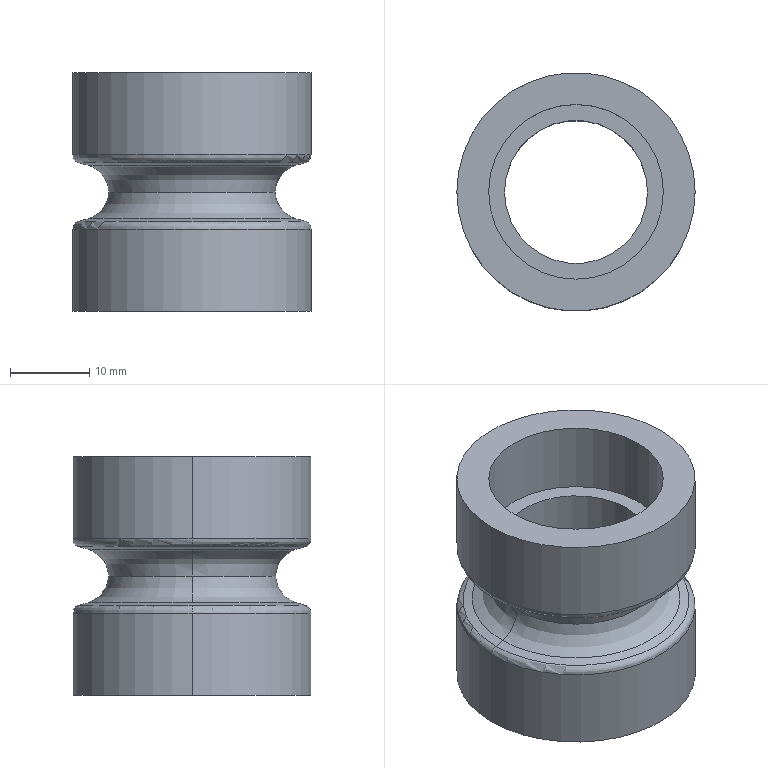Component | SolidWorks | JL001-03-03-1_JL001-03-03-002-1 | 1 solid | 26 faces | box 30 x 30 x 30 mm | volume 9084 mm3 | cylinder 10 | torus 8 | cone 4 | plane 4 | commonest cylinder face diameters 22 x4 30 x4 18 x2
build123d program:
from build123d import *

# Parameters (mm, degrees)
FILLET1_R = 1


with BuildPart() as part:
    # Sketch1 → Revolve1 (revolve)
    with BuildSketch(Plane.XY, mode=Mode.PRIVATE) as revolve1_sk:
        Polygon((11, 15), (15, 15), (15, -15), (11, -15), (11, -6), (9, -6), (9, 6), (11, 6), align=None)
    revolve(revolve1_sk.sketch.rotate(Axis((0, 0, 0), (0, -1, 0)), 90), axis=Axis((0, 0, 0), (0, -1, 0)))

    # Sketch2 → Cut-Revolve1 (revolve, cut)
    with BuildSketch(Plane.XY, mode=Mode.PRIVATE) as cut_revolve1_sk:
        with BuildLine():
            Line((13.094, 3.381), (16, 4.159))
            Line((16, 4.159), (16, -4.159))
            Line((16, -4.159), (13.094, -3.381))
            ThreePointArc((13.094, -3.381), (10.5, 0), (13.094, 3.381))
        make_face()
    revolve(cut_revolve1_sk.sketch.rotate(Axis((0, 0, 0), (0, -1, 0)), 90), axis=Axis((0, 0, 0), (0, -1, 0)), mode=Mode.SUBTRACT)

    # Fillet1
    fillet1_edges = [part.edges().sort_by_distance(p)[0] for p in [
        (0, -3.891, -15),
        (0, 3.891, -15),
    ]]
    fillet(fillet1_edges, radius=FILLET1_R)


solid = part.part

# Placed as in the assembly
solid = solid.moved(Location((15, 27.5, 40.5), (90, 0, 0)))
STEP:
#1=COLOUR_RGB('',0.7922,0.8196,0.9333);
#2=FILL_AREA_STYLE_COLOUR('',#1);
#3=FILL_AREA_STYLE('',(#2));
#4=SURFACE_STYLE_FILL_AREA(#3);
#5=SURFACE_SIDE_STYLE('',(#4));
#6=SURFACE_STYLE_USAGE(.BOTH.,#5);
#7=PRESENTATION_STYLE_ASSIGNMENT((#6));
#8=CARTESIAN_POINT('',(0.07503,1.083,1.728));
#9=VERTEX_POINT('',#8);
#10=CARTESIAN_POINT('',(0.1772,1.083,1.594));
#11=VERTEX_POINT('',#10);
#12=CARTESIAN_POINT('',(0.03937,1.083,1.594));
#13=DIRECTION('',(-0.,1.,0.));
#14=DIRECTION('',(-1.,0.,0.));
#15=AXIS2_PLACEMENT_3D('',#12,#13,#14);
#16=CIRCLE('',#15,0.1378);
#17=EDGE_CURVE('',#9,#11,#16,.T.);
#18=ORIENTED_EDGE('',*,*,#17,.T.);
#19=CARTESIAN_POINT('',(1.004,1.083,1.594));
#20=VERTEX_POINT('',#19);
#21=CARTESIAN_POINT('',(0.5906,1.083,1.594));
#22=DIRECTION('',(0.,0.,1.));
#23=DIRECTION('',(1.,0.,0.));
#24=AXIS2_PLACEMENT_3D('',#21,#22,#23);
#25=CIRCLE('',#24,0.4134);
#26=EDGE_CURVE('',#11,#20,#25,.T.);
#27=ORIENTED_EDGE('',*,*,#26,.T.);
#28=CARTESIAN_POINT('',(1.106,1.083,1.728));
#29=VERTEX_POINT('',#28);
#30=CARTESIAN_POINT('',(1.142,1.083,1.594));
#31=DIRECTION('',(0.,-1.,0.));
#32=DIRECTION('',(1.,0.,0.));
#33=AXIS2_PLACEMENT_3D('',#30,#31,#32);
#34=CIRCLE('',#33,0.1378);
#35=EDGE_CURVE('',#29,#20,#34,.T.);
#36=ORIENTED_EDGE('',*,*,#35,.F.);
#37=CARTESIAN_POINT('',(0.5906,1.083,1.728));
#38=DIRECTION('',(0.,0.,1.));
#39=DIRECTION('',(-1.,-0.,0.));
#40=AXIS2_PLACEMENT_3D('',#37,#38,#39);
#41=CIRCLE('',#40,0.5155);
#42=EDGE_CURVE('',#9,#29,#41,.T.);
#43=ORIENTED_EDGE('',*,*,#42,.F.);
#44=EDGE_LOOP('',(#18,#27,#36,#43));
#45=FACE_OUTER_BOUND('',#44,.T.);
#46=CARTESIAN_POINT('',(0.5906,1.083,1.594));
#47=DIRECTION('',(0.,0.,1.));
#48=DIRECTION('',(-1.,-0.,0.));
#49=AXIS2_PLACEMENT_3D('',#46,#47,#48);
#50=TOROIDAL_SURFACE('',#49,0.5512,0.1378);
#51=ADVANCED_FACE('',(#45),#50,.F.);
#52=ORIENTED_EDGE('',*,*,#35,.T.);
#53=CARTESIAN_POINT('',(0.5906,1.083,1.594));
#54=DIRECTION('',(0.,0.,1.));
#55=DIRECTION('',(1.,0.,0.));
#56=AXIS2_PLACEMENT_3D('',#53,#54,#55);
#57=CIRCLE('',#56,0.4134);
#58=EDGE_CURVE('',#20,#11,#57,.T.);
#59=ORIENTED_EDGE('',*,*,#58,.T.);
#60=ORIENTED_EDGE('',*,*,#17,.F.);
#61=CARTESIAN_POINT('',(0.5906,1.083,1.728));
#62=DIRECTION('',(0.,0.,1.));
#63=DIRECTION('',(-1.,-0.,0.));
#64=AXIS2_PLACEMENT_3D('',#61,#62,#63);
#65=CIRCLE('',#64,0.5155);
#66=EDGE_CURVE('',#29,#9,#65,.T.);
#67=ORIENTED_EDGE('',*,*,#66,.F.);
#68=EDGE_LOOP('',(#52,#59,#60,#67));
#69=FACE_OUTER_BOUND('',#68,.T.);
#70=CARTESIAN_POINT('',(0.5906,1.083,1.594));
#71=DIRECTION('',(0.,0.,1.));
#72=DIRECTION('',(-1.,-0.,0.));
#73=AXIS2_PLACEMENT_3D('',#70,#71,#72);
#74=TOROIDAL_SURFACE('',#73,0.5512,0.1378);
#75=ADVANCED_FACE('',(#69),#74,.F.);
#76=CARTESIAN_POINT('',(1.152,1.083,1.74));
#77=VERTEX_POINT('',#76);
#78=CARTESIAN_POINT('',(0.02918,1.083,1.74));
#79=VERTEX_POINT('',#78);
#80=CARTESIAN_POINT('',(0.5906,1.083,1.74));
#81=DIRECTION('',(0.,0.,-1.));
#82=DIRECTION('',(-1.,-0.,0.));
#83=AXIS2_PLACEMENT_3D('',#80,#81,#82);
#84=CIRCLE('',#83,0.5614);
#85=EDGE_CURVE('',#77,#79,#84,.T.);
#86=ORIENTED_EDGE('',*,*,#85,.F.);
#87=CARTESIAN_POINT('',(1.181,1.083,1.778));
#88=VERTEX_POINT('',#87);
#89=CARTESIAN_POINT('',(1.142,1.083,1.778));
#90=DIRECTION('',(0.,-1.,0.));
#91=DIRECTION('',(1.,0.,0.));
#92=AXIS2_PLACEMENT_3D('',#89,#90,#91);
#93=CIRCLE('',#92,0.03937);
#94=EDGE_CURVE('',#77,#88,#93,.T.);
#95=ORIENTED_EDGE('',*,*,#94,.T.);
#96=CARTESIAN_POINT('',(-0.,1.083,1.778));
#97=VERTEX_POINT('',#96);
#98=CARTESIAN_POINT('',(0.5906,1.083,1.778));
#99=DIRECTION('',(0.,0.,1.));
#100=DIRECTION('',(-1.,-0.,0.));
#101=AXIS2_PLACEMENT_3D('',#98,#99,#100);
#102=CIRCLE('',#101,0.5906);
#103=EDGE_CURVE('',#97,#88,#102,.T.);
#104=ORIENTED_EDGE('',*,*,#103,.F.);
#105=CARTESIAN_POINT('',(0.03937,1.083,1.778));
#106=DIRECTION('',(-0.,1.,0.));
#107=DIRECTION('',(-1.,0.,0.));
#108=AXIS2_PLACEMENT_3D('',#105,#106,#107);
#109=CIRCLE('',#108,0.03937);
#110=EDGE_CURVE('',#79,#97,#109,.T.);
#111=ORIENTED_EDGE('',*,*,#110,.F.);
#112=EDGE_LOOP('',(#86,#95,#104,#111));
#113=FACE_OUTER_BOUND('',#112,.T.);
#114=CARTESIAN_POINT('',(0.5906,1.083,1.778));
#115=DIRECTION('',(0.,0.,1.));
#116=DIRECTION('',(-1.,-0.,0.));
#117=AXIS2_PLACEMENT_3D('',#114,#115,#116);
#118=TOROIDAL_SURFACE('',#117,0.5512,0.03937);
#119=ADVANCED_FACE('',(#113),#118,.T.);
#120=CARTESIAN_POINT('',(0.02918,1.083,1.449));
#121=VERTEX_POINT('',#120);
#122=CARTESIAN_POINT('',(1.152,1.083,1.449));
#123=VERTEX_POINT('',#122);
#124=CARTESIAN_POINT('',(0.5906,1.083,1.449));
#125=DIRECTION('',(0.,0.,1.));
#126=DIRECTION('',(1.,0.,0.));
#127=AXIS2_PLACEMENT_3D('',#124,#125,#126);
#128=CIRCLE('',#127,0.5614);
#129=EDGE_CURVE('',#121,#123,#128,.T.);
#130=ORIENTED_EDGE('',*,*,#129,.F.);
#131=CARTESIAN_POINT('',(-0.,1.083,1.411));
#132=VERTEX_POINT('',#131);
#133=CARTESIAN_POINT('',(0.03937,1.083,1.411));
#134=DIRECTION('',(0.,-1.,0.));
#135=DIRECTION('',(1.,0.,0.));
#136=AXIS2_PLACEMENT_3D('',#133,#134,#135);
#137=CIRCLE('',#136,0.03937);
#138=EDGE_CURVE('',#121,#132,#137,.T.);
#139=ORIENTED_EDGE('',*,*,#138,.T.);
#140=CARTESIAN_POINT('',(1.181,1.083,1.411));
#141=VERTEX_POINT('',#140);
#142=CARTESIAN_POINT('',(0.5906,1.083,1.411));
#143=DIRECTION('',(0.,0.,-1.));
#144=DIRECTION('',(1.,0.,0.));
#145=AXIS2_PLACEMENT_3D('',#142,#143,#144);
#146=CIRCLE('',#145,0.5906);
#147=EDGE_CURVE('',#141,#132,#146,.T.);
#148=ORIENTED_EDGE('',*,*,#147,.F.);
#149=CARTESIAN_POINT('',(1.142,1.083,1.411));
#150=DIRECTION('',(-0.,1.,0.));
#151=DIRECTION('',(-1.,0.,0.));
#152=AXIS2_PLACEMENT_3D('',#149,#150,#151);
#153=CIRCLE('',#152,0.03937);
#154=EDGE_CURVE('',#123,#141,#153,.T.);
#155=ORIENTED_EDGE('',*,*,#154,.F.);
#156=EDGE_LOOP('',(#130,#139,#148,#155));
#157=FACE_OUTER_BOUND('',#156,.T.);
#158=CARTESIAN_POINT('',(0.5906,1.083,1.411));
#159=DIRECTION('',(0.,0.,-1.));
#160=DIRECTION('',(1.,0.,0.));
#161=AXIS2_PLACEMENT_3D('',#158,#159,#160);
#162=TOROIDAL_SURFACE('',#161,0.5512,0.03937);
#163=ADVANCED_FACE('',(#157),#162,.T.);
#164=ORIENTED_EDGE('',*,*,#58,.F.);
#165=CARTESIAN_POINT('',(1.106,1.083,1.461));
#166=VERTEX_POINT('',#165);
#167=CARTESIAN_POINT('',(1.142,1.083,1.594));
#168=DIRECTION('',(0.,-1.,0.));
#169=DIRECTION('',(1.,0.,0.));
#170=AXIS2_PLACEMENT_3D('',#167,#168,#169);
#171=CIRCLE('',#170,0.1378);
#172=EDGE_CURVE('',#20,#166,#171,.T.);
#173=ORIENTED_EDGE('',*,*,#172,.T.);
#174=CARTESIAN_POINT('',(0.07503,1.083,1.461));
#175=VERTEX_POINT('',#174);
#176=CARTESIAN_POINT('',(0.5906,1.083,1.461));
#177=DIRECTION('',(0.,0.,1.));
#178=DIRECTION('',(-1.,-0.,0.));
#179=AXIS2_PLACEMENT_3D('',#176,#177,#178);
#180=CIRCLE('',#179,0.5155);
#181=EDGE_CURVE('',#166,#175,#180,.T.);
#182=ORIENTED_EDGE('',*,*,#181,.T.);
#183=CARTESIAN_POINT('',(0.03937,1.083,1.594));
#184=DIRECTION('',(-0.,1.,0.));
#185=DIRECTION('',(-1.,0.,0.));
#186=AXIS2_PLACEMENT_3D('',#183,#184,#185);
#187=CIRCLE('',#186,0.1378);
#188=EDGE_CURVE('',#11,#175,#187,.T.);
#189=ORIENTED_EDGE('',*,*,#188,.F.);
#190=EDGE_LOOP('',(#164,#173,#182,#189));
#191=FACE_OUTER_BOUND('',#190,.T.);
#192=CARTESIAN_POINT('',(0.5906,1.083,1.594));
#193=DIRECTION('',(0.,0.,1.));
#194=DIRECTION('',(-1.,-0.,0.));
#195=AXIS2_PLACEMENT_3D('',#192,#193,#194);
#196=TOROIDAL_SURFACE('',#195,0.5512,0.1378);
#197=ADVANCED_FACE('',(#191),#196,.F.);
#198=ORIENTED_EDGE('',*,*,#42,.T.);
#199=CARTESIAN_POINT('',(1.22,1.083,1.758));
#200=DIRECTION('',(0.9659,0.,0.2588));
#201=VECTOR('',#200,39.37);
#202=LINE('',#199,#201);
#203=EDGE_CURVE('',#29,#77,#202,.T.);
#204=ORIENTED_EDGE('',*,*,#203,.T.);
#205=ORIENTED_EDGE('',*,*,#85,.T.);
#206=CARTESIAN_POINT('',(-0.03937,1.083,1.758));
#207=DIRECTION('',(-0.9659,-0.,0.2588));
#208=VECTOR('',#207,39.37);
#209=LINE('',#206,#208);
#210=EDGE_CURVE('',#9,#79,#209,.T.);
#211=ORIENTED_EDGE('',*,*,#210,.F.);
#212=EDGE_LOOP('',(#198,#204,#205,#211));
#213=FACE_OUTER_BOUND('',#212,.T.);
#214=CARTESIAN_POINT('',(0.5906,1.083,1.758));
#215=DIRECTION('',(0.,0.,1.));
#216=DIRECTION('',(-1.,-0.,0.));
#217=AXIS2_PLACEMENT_3D('',#214,#215,#216);
#218=CONICAL_SURFACE('',#217,0.6299,1.309);
#219=ADVANCED_FACE('',(#213),#218,.T.);
#220=CARTESIAN_POINT('',(0.5906,1.083,1.461));
#221=DIRECTION('',(0.,0.,1.));
#222=DIRECTION('',(-1.,-0.,0.));
#223=AXIS2_PLACEMENT_3D('',#220,#221,#222);
#224=CIRCLE('',#223,0.5155);
#225=EDGE_CURVE('',#175,#166,#224,.T.);
#226=ORIENTED_EDGE('',*,*,#225,.F.);
#227=CARTESIAN_POINT('',(0.07503,1.083,1.461));
#228=DIRECTION('',(-0.9659,-0.,-0.2588));
#229=VECTOR('',#228,39.37);
#230=LINE('',#227,#229);
#231=EDGE_CURVE('',#175,#121,#230,.T.);
#232=ORIENTED_EDGE('',*,*,#231,.T.);
#233=ORIENTED_EDGE('',*,*,#129,.T.);
#234=CARTESIAN_POINT('',(1.106,1.083,1.461));
#235=DIRECTION('',(0.9659,0.,-0.2588));
#236=VECTOR('',#235,39.37);
#237=LINE('',#234,#236);
#238=EDGE_CURVE('',#166,#123,#237,.T.);
#239=ORIENTED_EDGE('',*,*,#238,.F.);
#240=EDGE_LOOP('',(#226,#232,#233,#239));
#241=FACE_OUTER_BOUND('',#240,.T.);
#242=CARTESIAN_POINT('',(0.5906,1.083,1.461));
#243=DIRECTION('',(0.,0.,-1.));
#244=DIRECTION('',(1.,0.,0.));
#245=AXIS2_PLACEMENT_3D('',#242,#243,#244);
#246=CONICAL_SURFACE('',#245,0.5155,1.309);
#247=ADVANCED_FACE('',(#241),#246,.T.);
#248=CARTESIAN_POINT('',(0.9449,1.083,1.358));
#249=VERTEX_POINT('',#248);
#250=CARTESIAN_POINT('',(0.2362,1.083,1.358));
#251=VERTEX_POINT('',#250);
#252=CARTESIAN_POINT('',(0.5906,1.083,1.358));
#253=DIRECTION('',(0.,0.,1.));
#254=DIRECTION('',(-1.,-0.,0.));
#255=AXIS2_PLACEMENT_3D('',#252,#253,#254);
#256=CIRCLE('',#255,0.3543);
#257=EDGE_CURVE('',#249,#251,#256,.T.);
#258=ORIENTED_EDGE('',*,*,#257,.F.);
#259=CARTESIAN_POINT('',(0.9449,1.083,1.831));
#260=VERTEX_POINT('',#259);
#261=CARTESIAN_POINT('',(0.9449,1.083,1.594));
#262=DIRECTION('',(0.,0.,1.));
#263=VECTOR('',#262,39.37);
#264=LINE('',#261,#263);
#265=EDGE_CURVE('',#249,#260,#264,.T.);
#266=ORIENTED_EDGE('',*,*,#265,.T.);
#267=CARTESIAN_POINT('',(0.2362,1.083,1.831));
#268=VERTEX_POINT('',#267);
#269=CARTESIAN_POINT('',(0.5906,1.083,1.831));
#270=DIRECTION('',(0.,0.,1.));
#271=DIRECTION('',(-1.,-0.,0.));
#272=AXIS2_PLACEMENT_3D('',#269,#270,#271);
#273=CIRCLE('',#272,0.3543);
#274=EDGE_CURVE('',#260,#268,#273,.T.);
#275=ORIENTED_EDGE('',*,*,#274,.T.);
#276=CARTESIAN_POINT('',(0.2362,1.083,1.594));
#277=DIRECTION('',(0.,0.,1.));
#278=VECTOR('',#277,39.37);
#279=LINE('',#276,#278);
#280=EDGE_CURVE('',#251,#268,#279,.T.);
#281=ORIENTED_EDGE('',*,*,#280,.F.);
#282=EDGE_LOOP('',(#258,#266,#275,#281));
#283=FACE_OUTER_BOUND('',#282,.T.);
#284=CARTESIAN_POINT('',(0.5906,1.083,1.594));
#285=DIRECTION('',(0.,0.,1.));
#286=DIRECTION('',(-1.,-0.,0.));
#287=AXIS2_PLACEMENT_3D('',#284,#285,#286);
#288=CYLINDRICAL_SURFACE('',#287,0.3543);
#289=ADVANCED_FACE('',(#283),#288,.F.);
#290=CARTESIAN_POINT('',(1.024,1.083,1.004));
#291=VERTEX_POINT('',#290);
#292=CARTESIAN_POINT('',(0.1575,1.083,1.004));
#293=VERTEX_POINT('',#292);
#294=CARTESIAN_POINT('',(0.5906,1.083,1.004));
#295=DIRECTION('',(0.,0.,1.));
#296=DIRECTION('',(-1.,-0.,0.));
#297=AXIS2_PLACEMENT_3D('',#294,#295,#296);
#298=CIRCLE('',#297,0.4331);
#299=EDGE_CURVE('',#291,#293,#298,.T.);
#300=ORIENTED_EDGE('',*,*,#299,.F.);
#301=CARTESIAN_POINT('',(1.024,1.083,1.358));
#302=VERTEX_POINT('',#301);
#303=CARTESIAN_POINT('',(1.024,1.083,1.594));
#304=DIRECTION('',(0.,0.,1.));
#305=VECTOR('',#304,39.37);
#306=LINE('',#303,#305);
#307=EDGE_CURVE('',#291,#302,#306,.T.);
#308=ORIENTED_EDGE('',*,*,#307,.T.);
#309=CARTESIAN_POINT('',(0.1575,1.083,1.358));
#310=VERTEX_POINT('',#309);
#311=CARTESIAN_POINT('',(0.5906,1.083,1.358));
#312=DIRECTION('',(0.,0.,1.));
#313=DIRECTION('',(-1.,-0.,0.));
#314=AXIS2_PLACEMENT_3D('',#311,#312,#313);
#315=CIRCLE('',#314,0.4331);
#316=EDGE_CURVE('',#302,#310,#315,.T.);
#317=ORIENTED_EDGE('',*,*,#316,.T.);
#318=CARTESIAN_POINT('',(0.1575,1.083,1.594));
#319=DIRECTION('',(0.,0.,1.));
#320=VECTOR('',#319,39.37);
#321=LINE('',#318,#320);
#322=EDGE_CURVE('',#293,#310,#321,.T.);
#323=ORIENTED_EDGE('',*,*,#322,.F.);
#324=EDGE_LOOP('',(#300,#308,#317,#323));
#325=FACE_OUTER_BOUND('',#324,.T.);
#326=CARTESIAN_POINT('',(0.5906,1.083,1.594));
#327=DIRECTION('',(0.,0.,1.));
#328=DIRECTION('',(-1.,-0.,0.));
#329=AXIS2_PLACEMENT_3D('',#326,#327,#328);
#330=CYLINDRICAL_SURFACE('',#329,0.4331);
#331=ADVANCED_FACE('',(#325),#330,.F.);
#332=CARTESIAN_POINT('',(1.024,1.083,1.831));
#333=VERTEX_POINT('',#332);
#334=CARTESIAN_POINT('',(0.1575,1.083,1.831));
#335=VERTEX_POINT('',#334);
#336=CARTESIAN_POINT('',(0.5906,1.083,1.831));
#337=DIRECTION('',(0.,0.,1.));
#338=DIRECTION('',(-1.,-0.,0.));
#339=AXIS2_PLACEMENT_3D('',#336,#337,#338);
#340=CIRCLE('',#339,0.4331);
#341=EDGE_CURVE('',#333,#335,#340,.T.);
#342=ORIENTED_EDGE('',*,*,#341,.F.);
#343=CARTESIAN_POINT('',(1.024,1.083,2.185));
#344=VERTEX_POINT('',#343);
#345=CARTESIAN_POINT('',(1.024,1.083,1.594));
#346=DIRECTION('',(0.,0.,1.));
#347=VECTOR('',#346,39.37);
#348=LINE('',#345,#347);
#349=EDGE_CURVE('',#333,#344,#348,.T.);
#350=ORIENTED_EDGE('',*,*,#349,.T.);
#351=CARTESIAN_POINT('',(0.1575,1.083,2.185));
#352=VERTEX_POINT('',#351);
#353=CARTESIAN_POINT('',(0.5906,1.083,2.185));
#354=DIRECTION('',(0.,0.,1.));
#355=DIRECTION('',(-1.,-0.,0.));
#356=AXIS2_PLACEMENT_3D('',#353,#354,#355);
#357=CIRCLE('',#356,0.4331);
#358=EDGE_CURVE('',#344,#352,#357,.T.);
#359=ORIENTED_EDGE('',*,*,#358,.T.);
#360=CARTESIAN_POINT('',(0.1575,1.083,1.594));
#361=DIRECTION('',(0.,0.,1.));
#362=VECTOR('',#361,39.37);
#363=LINE('',#360,#362);
#364=EDGE_CURVE('',#335,#352,#363,.T.);
#365=ORIENTED_EDGE('',*,*,#364,.F.);
#366=EDGE_LOOP('',(#342,#350,#359,#365));
#367=FACE_OUTER_BOUND('',#366,.T.);
#368=CARTESIAN_POINT('',(0.5906,1.083,1.594));
#369=DIRECTION('',(0.,0.,1.));
#370=DIRECTION('',(-1.,-0.,0.));
#371=AXIS2_PLACEMENT_3D('',#368,#369,#370);
#372=CYLINDRICAL_SURFACE('',#371,0.4331);
#373=ADVANCED_FACE('',(#367),#372,.F.);
#374=ORIENTED_EDGE('',*,*,#103,.T.);
#375=CARTESIAN_POINT('',(1.181,1.083,2.185));
#376=VERTEX_POINT('',#375);
#377=CARTESIAN_POINT('',(1.181,1.083,1.594));
#378=DIRECTION('',(0.,0.,1.));
#379=VECTOR('',#378,39.37);
#380=LINE('',#377,#379);
#381=EDGE_CURVE('',#88,#376,#380,.T.);
#382=ORIENTED_EDGE('',*,*,#381,.T.);
#383=CARTESIAN_POINT('',(-0.,1.083,2.185));
#384=VERTEX_POINT('',#383);
#385=CARTESIAN_POINT('',(0.5906,1.083,2.185));
#386=DIRECTION('',(0.,0.,1.));
#387=DIRECTION('',(-1.,-0.,0.));
#388=AXIS2_PLACEMENT_3D('',#385,#386,#387);
#389=CIRCLE('',#388,0.5906);
#390=EDGE_CURVE('',#384,#376,#389,.T.);
#391=ORIENTED_EDGE('',*,*,#390,.F.);
#392=CARTESIAN_POINT('',(-0.,1.083,1.594));
#393=DIRECTION('',(0.,0.,1.));
#394=VECTOR('',#393,39.37);
#395=LINE('',#392,#394);
#396=EDGE_CURVE('',#97,#384,#395,.T.);
#397=ORIENTED_EDGE('',*,*,#396,.F.);
#398=EDGE_LOOP('',(#374,#382,#391,#397));
#399=FACE_OUTER_BOUND('',#398,.T.);
#400=CARTESIAN_POINT('',(0.5906,1.083,1.594));
#401=DIRECTION('',(0.,0.,1.));
#402=DIRECTION('',(-1.,-0.,0.));
#403=AXIS2_PLACEMENT_3D('',#400,#401,#402);
#404=CYLINDRICAL_SURFACE('',#403,0.5906);
#405=ADVANCED_FACE('',(#399),#404,.T.);
#406=CARTESIAN_POINT('',(-0.,1.083,1.004));
#407=VERTEX_POINT('',#406);
#408=CARTESIAN_POINT('',(1.181,1.083,1.004));
#409=VERTEX_POINT('',#408);
#410=CARTESIAN_POINT('',(0.5906,1.083,1.004));
#411=DIRECTION('',(0.,0.,1.));
#412=DIRECTION('',(-1.,-0.,0.));
#413=AXIS2_PLACEMENT_3D('',#410,#411,#412);
#414=CIRCLE('',#413,0.5906);
#415=EDGE_CURVE('',#407,#409,#414,.T.);
#416=ORIENTED_EDGE('',*,*,#415,.T.);
#417=CARTESIAN_POINT('',(1.181,1.083,1.594));
#418=DIRECTION('',(0.,0.,1.));
#419=VECTOR('',#418,39.37);
#420=LINE('',#417,#419);
#421=EDGE_CURVE('',#409,#141,#420,.T.);
#422=ORIENTED_EDGE('',*,*,#421,.T.);
#423=ORIENTED_EDGE('',*,*,#147,.T.);
#424=CARTESIAN_POINT('',(-0.,1.083,1.594));
#425=DIRECTION('',(0.,0.,1.));
#426=VECTOR('',#425,39.37);
#427=LINE('',#424,#426);
#428=EDGE_CURVE('',#407,#132,#427,.T.);
#429=ORIENTED_EDGE('',*,*,#428,.F.);
#430=EDGE_LOOP('',(#416,#422,#423,#429));
#431=FACE_OUTER_BOUND('',#430,.T.);
#432=CARTESIAN_POINT('',(0.5906,1.083,1.594));
#433=DIRECTION('',(0.,0.,1.));
#434=DIRECTION('',(-1.,-0.,0.));
#435=AXIS2_PLACEMENT_3D('',#432,#433,#434);
#436=CYLINDRICAL_SURFACE('',#435,0.5906);
#437=ADVANCED_FACE('',(#431),#436,.T.);
#438=ORIENTED_EDGE('',*,*,#421,.F.);
#439=CARTESIAN_POINT('',(0.5906,1.083,1.004));
#440=DIRECTION('',(0.,0.,1.));
#441=DIRECTION('',(-1.,-0.,0.));
#442=AXIS2_PLACEMENT_3D('',#439,#440,#441);
#443=CIRCLE('',#442,0.5906);
#444=EDGE_CURVE('',#409,#407,#443,.T.);
#445=ORIENTED_EDGE('',*,*,#444,.T.);
#446=ORIENTED_EDGE('',*,*,#428,.T.);
#447=CARTESIAN_POINT('',(0.5906,1.083,1.411));
#448=DIRECTION('',(0.,0.,-1.));
#449=DIRECTION('',(1.,0.,0.));
#450=AXIS2_PLACEMENT_3D('',#447,#448,#449);
#451=CIRCLE('',#450,0.5906);
#452=EDGE_CURVE('',#132,#141,#451,.T.);
#453=ORIENTED_EDGE('',*,*,#452,.T.);
#454=EDGE_LOOP('',(#438,#445,#446,#453));
#455=FACE_OUTER_BOUND('',#454,.T.);
#456=CARTESIAN_POINT('',(0.5906,1.083,1.594));
#457=DIRECTION('',(0.,0.,1.));
#458=DIRECTION('',(-1.,-0.,0.));
#459=AXIS2_PLACEMENT_3D('',#456,#457,#458);
#460=CYLINDRICAL_SURFACE('',#459,0.5906);
#461=ADVANCED_FACE('',(#455),#460,.T.);
#462=ORIENTED_EDGE('',*,*,#381,.F.);
#463=CARTESIAN_POINT('',(0.5906,1.083,1.778));
#464=DIRECTION('',(0.,0.,1.));
#465=DIRECTION('',(-1.,-0.,0.));
#466=AXIS2_PLACEMENT_3D('',#463,#464,#465);
#467=CIRCLE('',#466,0.5906);
#468=EDGE_CURVE('',#88,#97,#467,.T.);
#469=ORIENTED_EDGE('',*,*,#468,.T.);
#470=ORIENTED_EDGE('',*,*,#396,.T.);
#471=CARTESIAN_POINT('',(0.5906,1.083,2.185));
#472=DIRECTION('',(0.,0.,1.));
#473=DIRECTION('',(-1.,-0.,0.));
#474=AXIS2_PLACEMENT_3D('',#471,#472,#473);
#475=CIRCLE('',#474,0.5906);
#476=EDGE_CURVE('',#376,#384,#475,.T.);
#477=ORIENTED_EDGE('',*,*,#476,.F.);
#478=EDGE_LOOP('',(#462,#469,#470,#477));
#479=FACE_OUTER_BOUND('',#478,.T.);
#480=CARTESIAN_POINT('',(0.5906,1.083,1.594));
#481=DIRECTION('',(0.,0.,1.));
#482=DIRECTION('',(-1.,-0.,0.));
#483=AXIS2_PLACEMENT_3D('',#480,#481,#482);
#484=CYLINDRICAL_SURFACE('',#483,0.5906);
#485=ADVANCED_FACE('',(#479),#484,.T.);
#486=ORIENTED_EDGE('',*,*,#349,.F.);
#487=CARTESIAN_POINT('',(0.5906,1.083,1.831));
#488=DIRECTION('',(0.,0.,1.));
#489=DIRECTION('',(-1.,-0.,0.));
#490=AXIS2_PLACEMENT_3D('',#487,#488,#489);
#491=CIRCLE('',#490,0.4331);
#492=EDGE_CURVE('',#335,#333,#491,.T.);
#493=ORIENTED_EDGE('',*,*,#492,.F.);
#494=ORIENTED_EDGE('',*,*,#364,.T.);
#495=CARTESIAN_POINT('',(0.5906,1.083,2.185));
#496=DIRECTION('',(0.,0.,1.));
#497=DIRECTION('',(-1.,-0.,0.));
#498=AXIS2_PLACEMENT_3D('',#495,#496,#497);
#499=CIRCLE('',#498,0.4331);
#500=EDGE_CURVE('',#352,#344,#499,.T.);
#501=ORIENTED_EDGE('',*,*,#500,.T.);
#502=EDGE_LOOP('',(#486,#493,#494,#501));
#503=FACE_OUTER_BOUND('',#502,.T.);
#504=CARTESIAN_POINT('',(0.5906,1.083,1.594));
#505=DIRECTION('',(0.,0.,1.));
#506=DIRECTION('',(-1.,-0.,0.));
#507=AXIS2_PLACEMENT_3D('',#504,#505,#506);
#508=CYLINDRICAL_SURFACE('',#507,0.4331);
#509=ADVANCED_FACE('',(#503),#508,.F.);
#510=ORIENTED_EDGE('',*,*,#500,.F.);
#511=ORIENTED_EDGE('',*,*,#358,.F.);
#512=EDGE_LOOP('',(#510,#511));
#513=FACE_BOUND('',#512,.T.);
#514=ORIENTED_EDGE('',*,*,#390,.T.);
#515=ORIENTED_EDGE('',*,*,#476,.T.);
#516=EDGE_LOOP('',(#514,#515));
#517=FACE_OUTER_BOUND('',#516,.T.);
#518=CARTESIAN_POINT('',(0.5906,0.6496,2.185));
#519=DIRECTION('',(0.,0.,-1.));
#520=DIRECTION('',(1.,0.,0.));
#521=AXIS2_PLACEMENT_3D('',#518,#519,#520);
#522=PLANE('',#521);
#523=ADVANCED_FACE('',(#513,#517),#522,.F.);
#524=ORIENTED_EDGE('',*,*,#415,.F.);
#525=ORIENTED_EDGE('',*,*,#444,.F.);
#526=EDGE_LOOP('',(#524,#525));
#527=FACE_OUTER_BOUND('',#526,.T.);
#528=CARTESIAN_POINT('',(0.5906,1.083,1.004));
#529=DIRECTION('',(0.,0.,1.));
#530=DIRECTION('',(-1.,-0.,0.));
#531=AXIS2_PLACEMENT_3D('',#528,#529,#530);
#532=CIRCLE('',#531,0.4331);
#533=EDGE_CURVE('',#293,#291,#532,.T.);
#534=ORIENTED_EDGE('',*,*,#533,.T.);
#535=ORIENTED_EDGE('',*,*,#299,.T.);
#536=EDGE_LOOP('',(#534,#535));
#537=FACE_BOUND('',#536,.T.);
#538=CARTESIAN_POINT('',(0.5906,0.4921,1.004));
#539=DIRECTION('',(0.,0.,1.));
#540=DIRECTION('',(-1.,-0.,0.));
#541=AXIS2_PLACEMENT_3D('',#538,#539,#540);
#542=PLANE('',#541);
#543=ADVANCED_FACE('',(#527,#537),#542,.F.);
#544=ORIENTED_EDGE('',*,*,#307,.F.);
#545=ORIENTED_EDGE('',*,*,#533,.F.);
#546=ORIENTED_EDGE('',*,*,#322,.T.);
#547=CARTESIAN_POINT('',(0.5906,1.083,1.358));
#548=DIRECTION('',(0.,0.,1.));
#549=DIRECTION('',(-1.,-0.,0.));
#550=AXIS2_PLACEMENT_3D('',#547,#548,#549);
#551=CIRCLE('',#550,0.4331);
#552=EDGE_CURVE('',#310,#302,#551,.T.);
#553=ORIENTED_EDGE('',*,*,#552,.T.);
#554=EDGE_LOOP('',(#544,#545,#546,#553));
#555=FACE_OUTER_BOUND('',#554,.T.);
#556=CARTESIAN_POINT('',(0.5906,1.083,1.594));
#557=DIRECTION('',(0.,0.,1.));
#558=DIRECTION('',(-1.,-0.,0.));
#559=AXIS2_PLACEMENT_3D('',#556,#557,#558);
#560=CYLINDRICAL_SURFACE('',#559,0.4331);
#561=ADVANCED_FACE('',(#555),#560,.F.);
#562=ORIENTED_EDGE('',*,*,#552,.F.);
#563=ORIENTED_EDGE('',*,*,#316,.F.);
#564=EDGE_LOOP('',(#562,#563));
#565=FACE_OUTER_BOUND('',#564,.T.);
#566=CARTESIAN_POINT('',(0.5906,1.083,1.358));
#567=DIRECTION('',(0.,0.,1.));
#568=DIRECTION('',(-1.,-0.,0.));
#569=AXIS2_PLACEMENT_3D('',#566,#567,#568);
#570=CIRCLE('',#569,0.3543);
#571=EDGE_CURVE('',#251,#249,#570,.T.);
#572=ORIENTED_EDGE('',*,*,#571,.T.);
#573=ORIENTED_EDGE('',*,*,#257,.T.);
#574=EDGE_LOOP('',(#572,#573));
#575=FACE_BOUND('',#574,.T.);
#576=CARTESIAN_POINT('',(0.5906,0.6496,1.358));
#577=DIRECTION('',(0.,0.,1.));
#578=DIRECTION('',(-1.,-0.,0.));
#579=AXIS2_PLACEMENT_3D('',#576,#577,#578);
#580=PLANE('',#579);
#581=ADVANCED_FACE('',(#565,#575),#580,.F.);
#582=ORIENTED_EDGE('',*,*,#265,.F.);
#583=ORIENTED_EDGE('',*,*,#571,.F.);
#584=ORIENTED_EDGE('',*,*,#280,.T.);
#585=CARTESIAN_POINT('',(0.5906,1.083,1.831));
#586=DIRECTION('',(0.,0.,1.));
#587=DIRECTION('',(-1.,-0.,0.));
#588=AXIS2_PLACEMENT_3D('',#585,#586,#587);
#589=CIRCLE('',#588,0.3543);
#590=EDGE_CURVE('',#268,#260,#589,.T.);
#591=ORIENTED_EDGE('',*,*,#590,.T.);
#592=EDGE_LOOP('',(#582,#583,#584,#591));
#593=FACE_OUTER_BOUND('',#592,.T.);
#594=CARTESIAN_POINT('',(0.5906,1.083,1.594));
#595=DIRECTION('',(0.,0.,1.));
#596=DIRECTION('',(-1.,-0.,0.));
#597=AXIS2_PLACEMENT_3D('',#594,#595,#596);
#598=CYLINDRICAL_SURFACE('',#597,0.3543);
#599=ADVANCED_FACE('',(#593),#598,.F.);
#600=ORIENTED_EDGE('',*,*,#590,.F.);
#601=ORIENTED_EDGE('',*,*,#274,.F.);
#602=EDGE_LOOP('',(#600,#601));
#603=FACE_BOUND('',#602,.T.);
#604=ORIENTED_EDGE('',*,*,#492,.T.);
#605=ORIENTED_EDGE('',*,*,#341,.T.);
#606=EDGE_LOOP('',(#604,#605));
#607=FACE_OUTER_BOUND('',#606,.T.);
#608=CARTESIAN_POINT('',(0.5906,0.7283,1.831));
#609=DIRECTION('',(0.,0.,-1.));
#610=DIRECTION('',(1.,0.,0.));
#611=AXIS2_PLACEMENT_3D('',#608,#609,#610);
#612=PLANE('',#611);
#613=ADVANCED_FACE('',(#603,#607),#612,.F.);
#614=ORIENTED_EDGE('',*,*,#231,.F.);
#615=ORIENTED_EDGE('',*,*,#181,.F.);
#616=ORIENTED_EDGE('',*,*,#238,.T.);
#617=CARTESIAN_POINT('',(0.5906,1.083,1.449));
#618=DIRECTION('',(0.,0.,1.));
#619=DIRECTION('',(1.,0.,0.));
#620=AXIS2_PLACEMENT_3D('',#617,#618,#619);
#621=CIRCLE('',#620,0.5614);
#622=EDGE_CURVE('',#123,#121,#621,.T.);
#623=ORIENTED_EDGE('',*,*,#622,.T.);
#624=EDGE_LOOP('',(#614,#615,#616,#623));
#625=FACE_OUTER_BOUND('',#624,.T.);
#626=CARTESIAN_POINT('',(0.5906,1.083,1.461));
#627=DIRECTION('',(0.,0.,-1.));
#628=DIRECTION('',(1.,0.,0.));
#629=AXIS2_PLACEMENT_3D('',#626,#627,#628);
#630=CONICAL_SURFACE('',#629,0.5155,1.309);
#631=ADVANCED_FACE('',(#625),#630,.T.);
#632=ORIENTED_EDGE('',*,*,#203,.F.);
#633=ORIENTED_EDGE('',*,*,#66,.T.);
#634=ORIENTED_EDGE('',*,*,#210,.T.);
#635=CARTESIAN_POINT('',(0.5906,1.083,1.74));
#636=DIRECTION('',(0.,0.,-1.));
#637=DIRECTION('',(-1.,-0.,0.));
#638=AXIS2_PLACEMENT_3D('',#635,#636,#637);
#639=CIRCLE('',#638,0.5614);
#640=EDGE_CURVE('',#79,#77,#639,.T.);
#641=ORIENTED_EDGE('',*,*,#640,.T.);
#642=EDGE_LOOP('',(#632,#633,#634,#641));
#643=FACE_OUTER_BOUND('',#642,.T.);
#644=CARTESIAN_POINT('',(0.5906,1.083,1.758));
#645=DIRECTION('',(0.,0.,1.));
#646=DIRECTION('',(-1.,-0.,0.));
#647=AXIS2_PLACEMENT_3D('',#644,#645,#646);
#648=CONICAL_SURFACE('',#647,0.6299,1.309);
#649=ADVANCED_FACE('',(#643),#648,.T.);
#650=ORIENTED_EDGE('',*,*,#26,.F.);
#651=ORIENTED_EDGE('',*,*,#188,.T.);
#652=ORIENTED_EDGE('',*,*,#225,.T.);
#653=ORIENTED_EDGE('',*,*,#172,.F.);
#654=EDGE_LOOP('',(#650,#651,#652,#653));
#655=FACE_OUTER_BOUND('',#654,.T.);
#656=CARTESIAN_POINT('',(0.5906,1.083,1.594));
#657=DIRECTION('',(0.,0.,1.));
#658=DIRECTION('',(-1.,-0.,0.));
#659=AXIS2_PLACEMENT_3D('',#656,#657,#658);
#660=TOROIDAL_SURFACE('',#659,0.5512,0.1378);
#661=ADVANCED_FACE('',(#655),#660,.F.);
#662=ORIENTED_EDGE('',*,*,#138,.F.);
#663=ORIENTED_EDGE('',*,*,#622,.F.);
#664=ORIENTED_EDGE('',*,*,#154,.T.);
#665=ORIENTED_EDGE('',*,*,#452,.F.);
#666=EDGE_LOOP('',(#662,#663,#664,#665));
#667=FACE_OUTER_BOUND('',#666,.T.);
#668=CARTESIAN_POINT('',(0.5906,1.083,1.411));
#669=DIRECTION('',(0.,0.,-1.));
#670=DIRECTION('',(1.,0.,0.));
#671=AXIS2_PLACEMENT_3D('',#668,#669,#670);
#672=TOROIDAL_SURFACE('',#671,0.5512,0.03937);
#673=ADVANCED_FACE('',(#667),#672,.T.);
#674=ORIENTED_EDGE('',*,*,#94,.F.);
#675=ORIENTED_EDGE('',*,*,#640,.F.);
#676=ORIENTED_EDGE('',*,*,#110,.T.);
#677=ORIENTED_EDGE('',*,*,#468,.F.);
#678=EDGE_LOOP('',(#674,#675,#676,#677));
#679=FACE_OUTER_BOUND('',#678,.T.);
#680=CARTESIAN_POINT('',(0.5906,1.083,1.778));
#681=DIRECTION('',(0.,0.,1.));
#682=DIRECTION('',(-1.,-0.,0.));
#683=AXIS2_PLACEMENT_3D('',#680,#681,#682);
#684=TOROIDAL_SURFACE('',#683,0.5512,0.03937);
#685=ADVANCED_FACE('',(#679),#684,.T.);
#686=CLOSED_SHELL('',(#51,#75,#119,#163,#197,#219,#247,#289,#331,#373,#405,#437,#461,#485,#509,#523,#543,#561,#581,#599,#613,#631,#649,#661,#673,#685));
#687=MANIFOLD_SOLID_BREP('',#686);
#688=STYLED_ITEM('',(#7),#687);
#689=PRESENTATION_LAYER_ASSIGNMENT('','',(#688));
#690=(LENGTH_UNIT()NAMED_UNIT(*)SI_UNIT($,.METRE.));
#691=LENGTH_MEASURE_WITH_UNIT(LENGTH_MEASURE(0.0254),#690);
#692=DIMENSIONAL_EXPONENTS(1.,0.,0.,0.,0.,0.,0.);
#693=(CONVERSION_BASED_UNIT('',#691)LENGTH_UNIT()NAMED_UNIT(#692));
#694=UNCERTAINTY_MEASURE_WITH_UNIT(LENGTH_MEASURE(0.00001),#693,'','');
#695=(NAMED_UNIT(*)PLANE_ANGLE_UNIT()SI_UNIT($,.RADIAN.));
#696=(NAMED_UNIT(*)SI_UNIT($,.STERADIAN.)SOLID_ANGLE_UNIT());
#697=(GEOMETRIC_REPRESENTATION_CONTEXT(3)GLOBAL_UNCERTAINTY_ASSIGNED_CONTEXT((#694))GLOBAL_UNIT_ASSIGNED_CONTEXT((#693,#695,#696))REPRESENTATION_CONTEXT('',''));
#698=MECHANICAL_DESIGN_GEOMETRIC_PRESENTATION_REPRESENTATION('',(#688),#697);
#699=CARTESIAN_POINT('',(0.,0.,0.));
#700=DIRECTION('',(0.,0.,1.));
#701=DIRECTION('',(1.,0.,0.));
#702=AXIS2_PLACEMENT_3D('',#699,#700,#701);
#703=(LENGTH_UNIT()NAMED_UNIT(*)SI_UNIT($,.METRE.));
#704=LENGTH_MEASURE_WITH_UNIT(LENGTH_MEASURE(0.0254),#703);
#705=DIMENSIONAL_EXPONENTS(1.,0.,0.,0.,0.,0.,0.);
#706=(CONVERSION_BASED_UNIT('',#704)LENGTH_UNIT()NAMED_UNIT(#705));
#707=UNCERTAINTY_MEASURE_WITH_UNIT(LENGTH_MEASURE(0.00001),#706,'','');
#708=(NAMED_UNIT(*)PLANE_ANGLE_UNIT()SI_UNIT($,.RADIAN.));
#709=(NAMED_UNIT(*)SI_UNIT($,.STERADIAN.)SOLID_ANGLE_UNIT());
#710=(GEOMETRIC_REPRESENTATION_CONTEXT(3)GLOBAL_UNCERTAINTY_ASSIGNED_CONTEXT((#707))GLOBAL_UNIT_ASSIGNED_CONTEXT((#706,#708,#709))REPRESENTATION_CONTEXT('',''));
#711=ADVANCED_BREP_SHAPE_REPRESENTATION('',(#687,#702),#710);